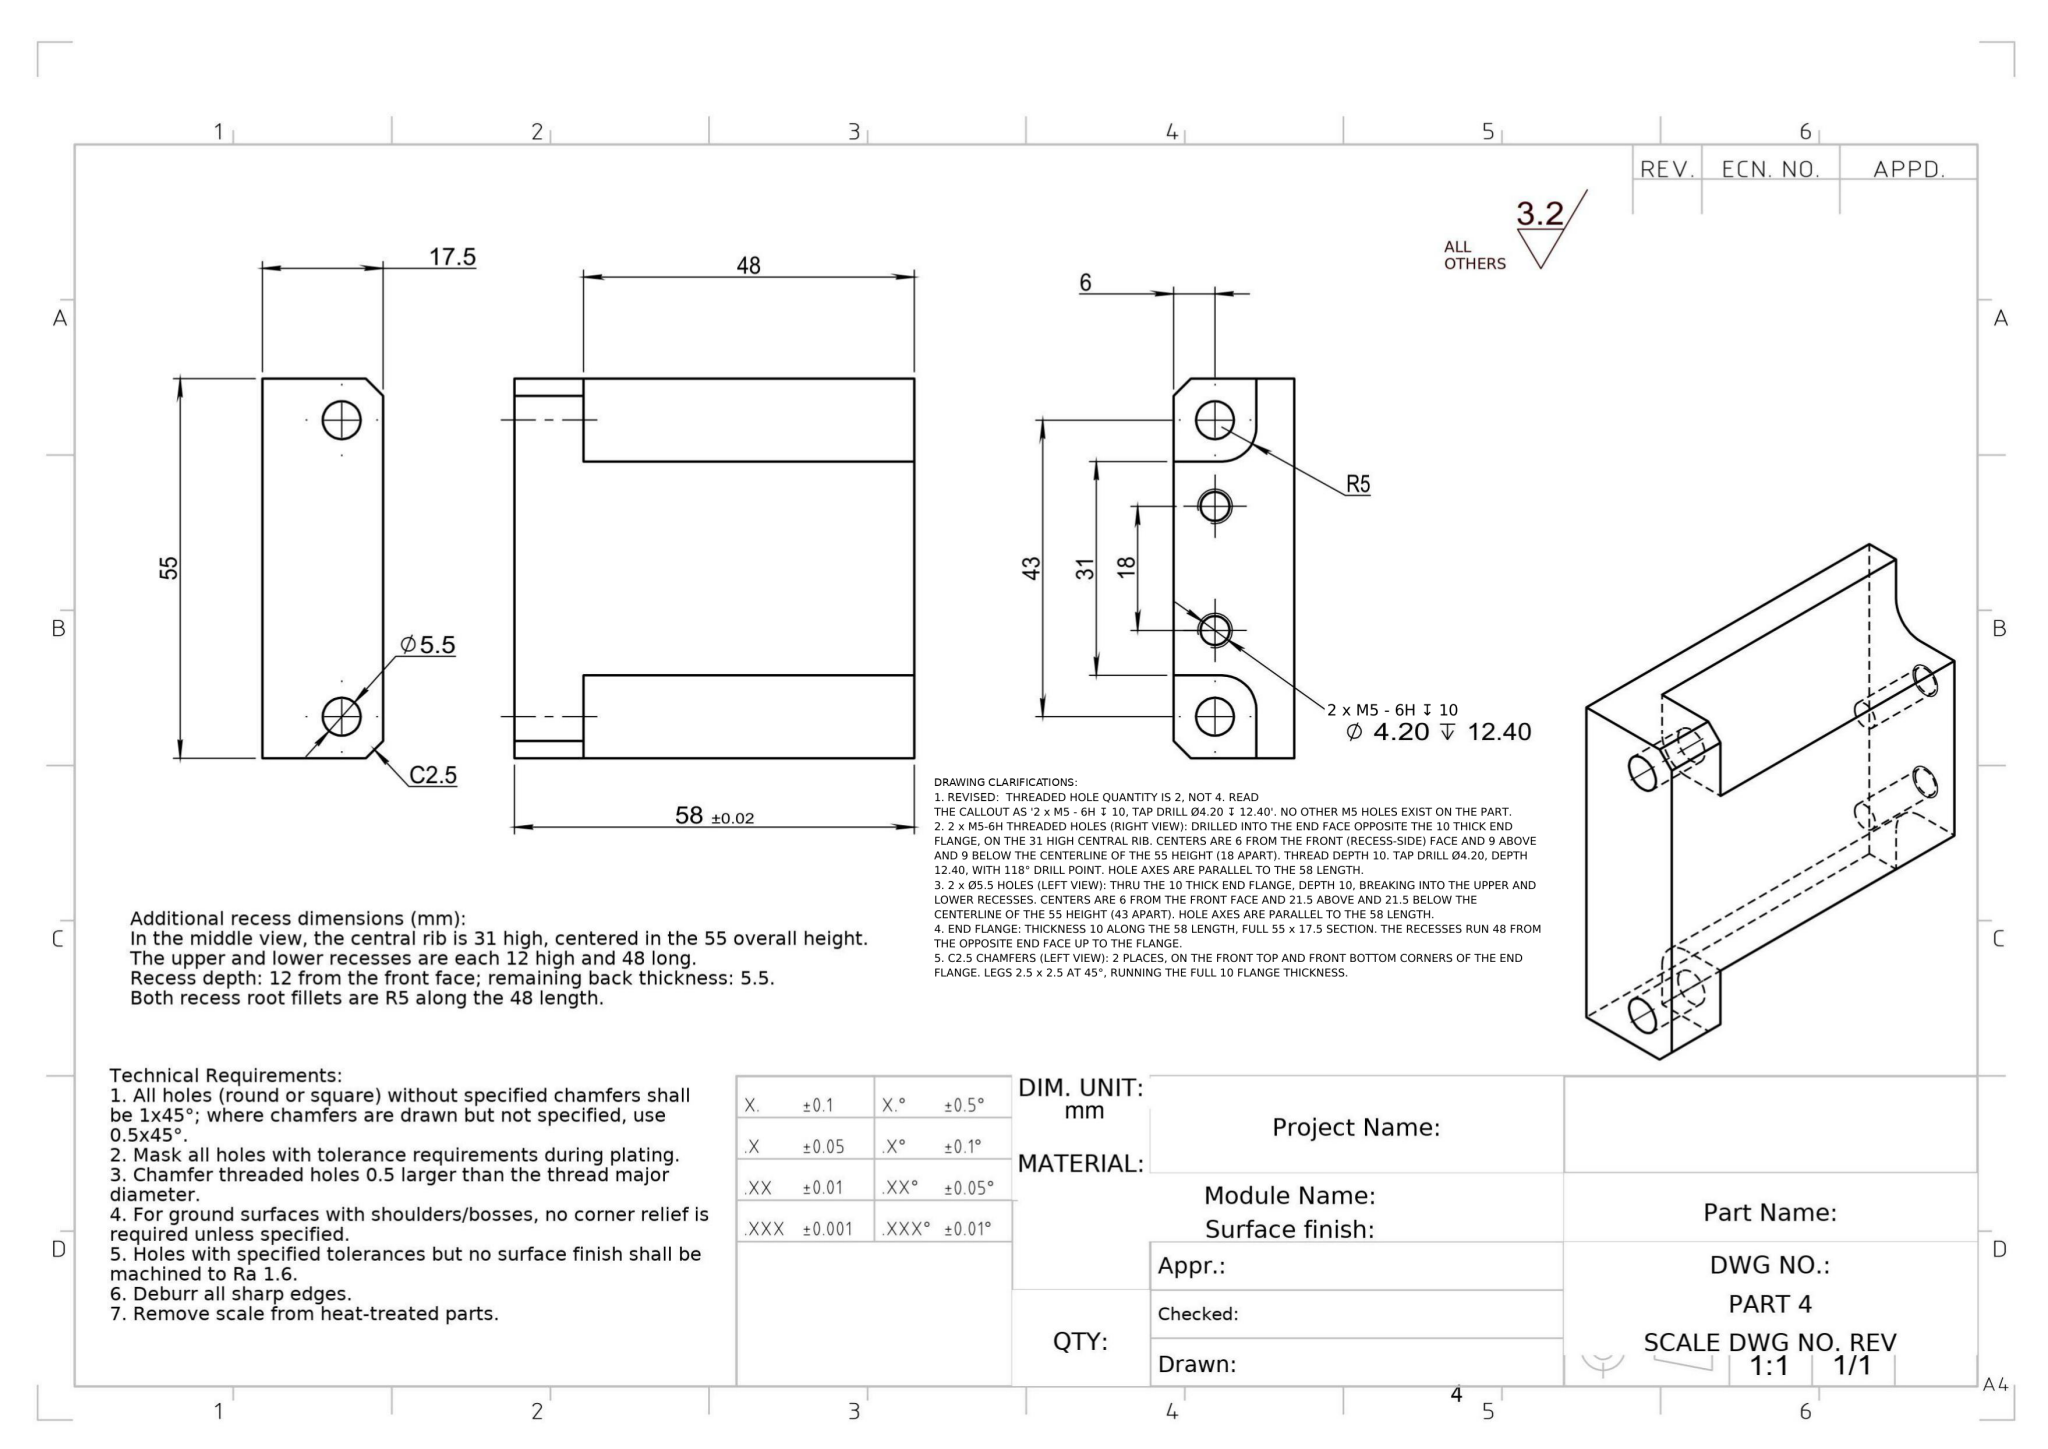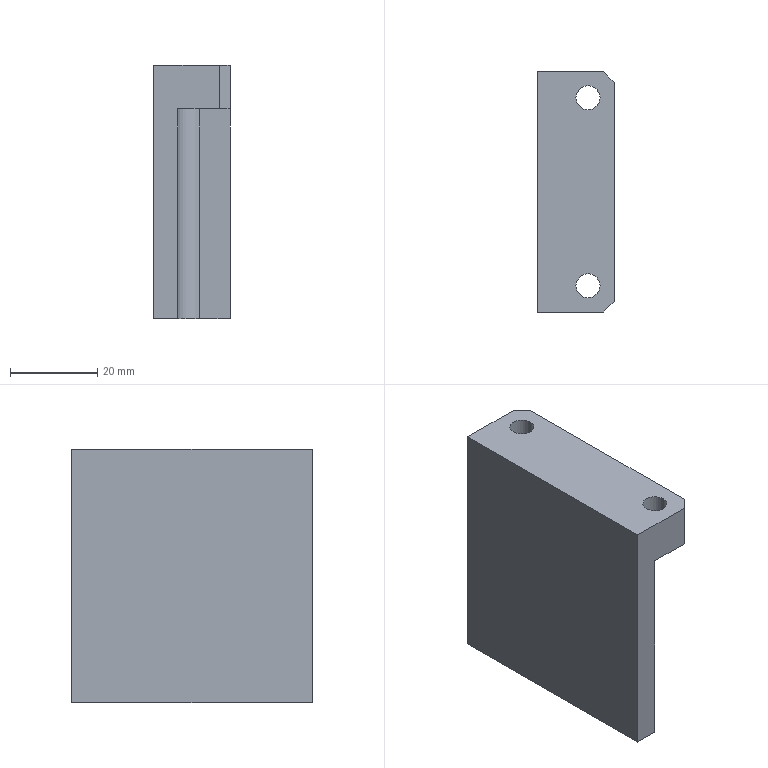Part | NX | mm | Grooved Vertical Mounting Block | 1 solid | 28 faces | box 17.5 x 55 x 58 mm | volume 41623 mm3 | plane 14 | cylinder 10 | cone 4 | commonest cylinder face diameters 4.2 x4 5.5 x4 10 x2